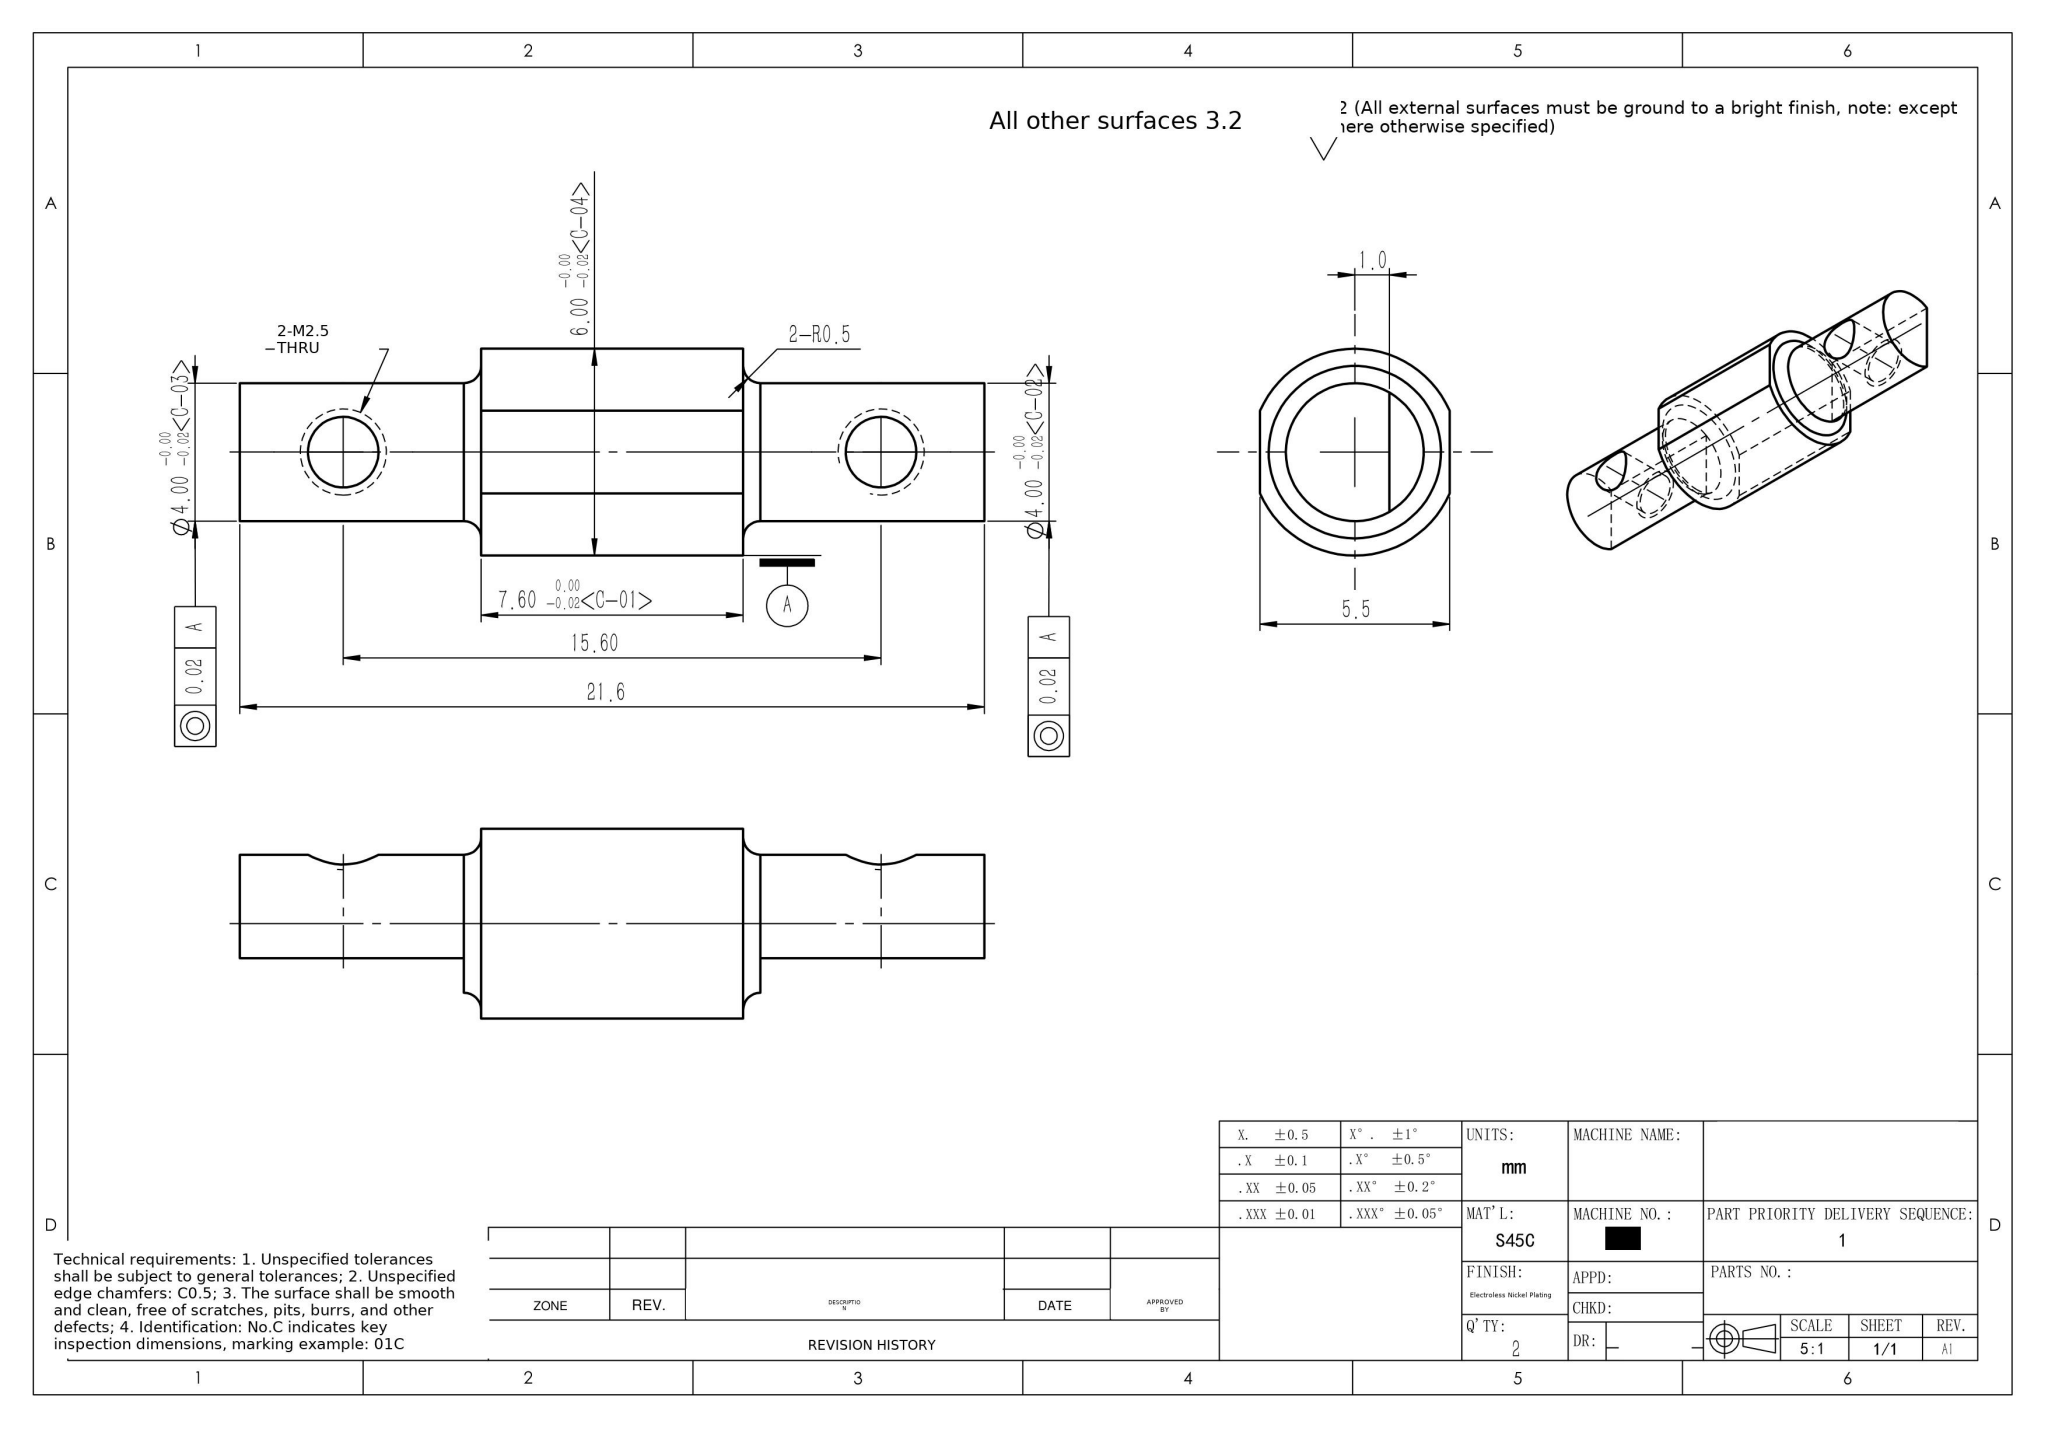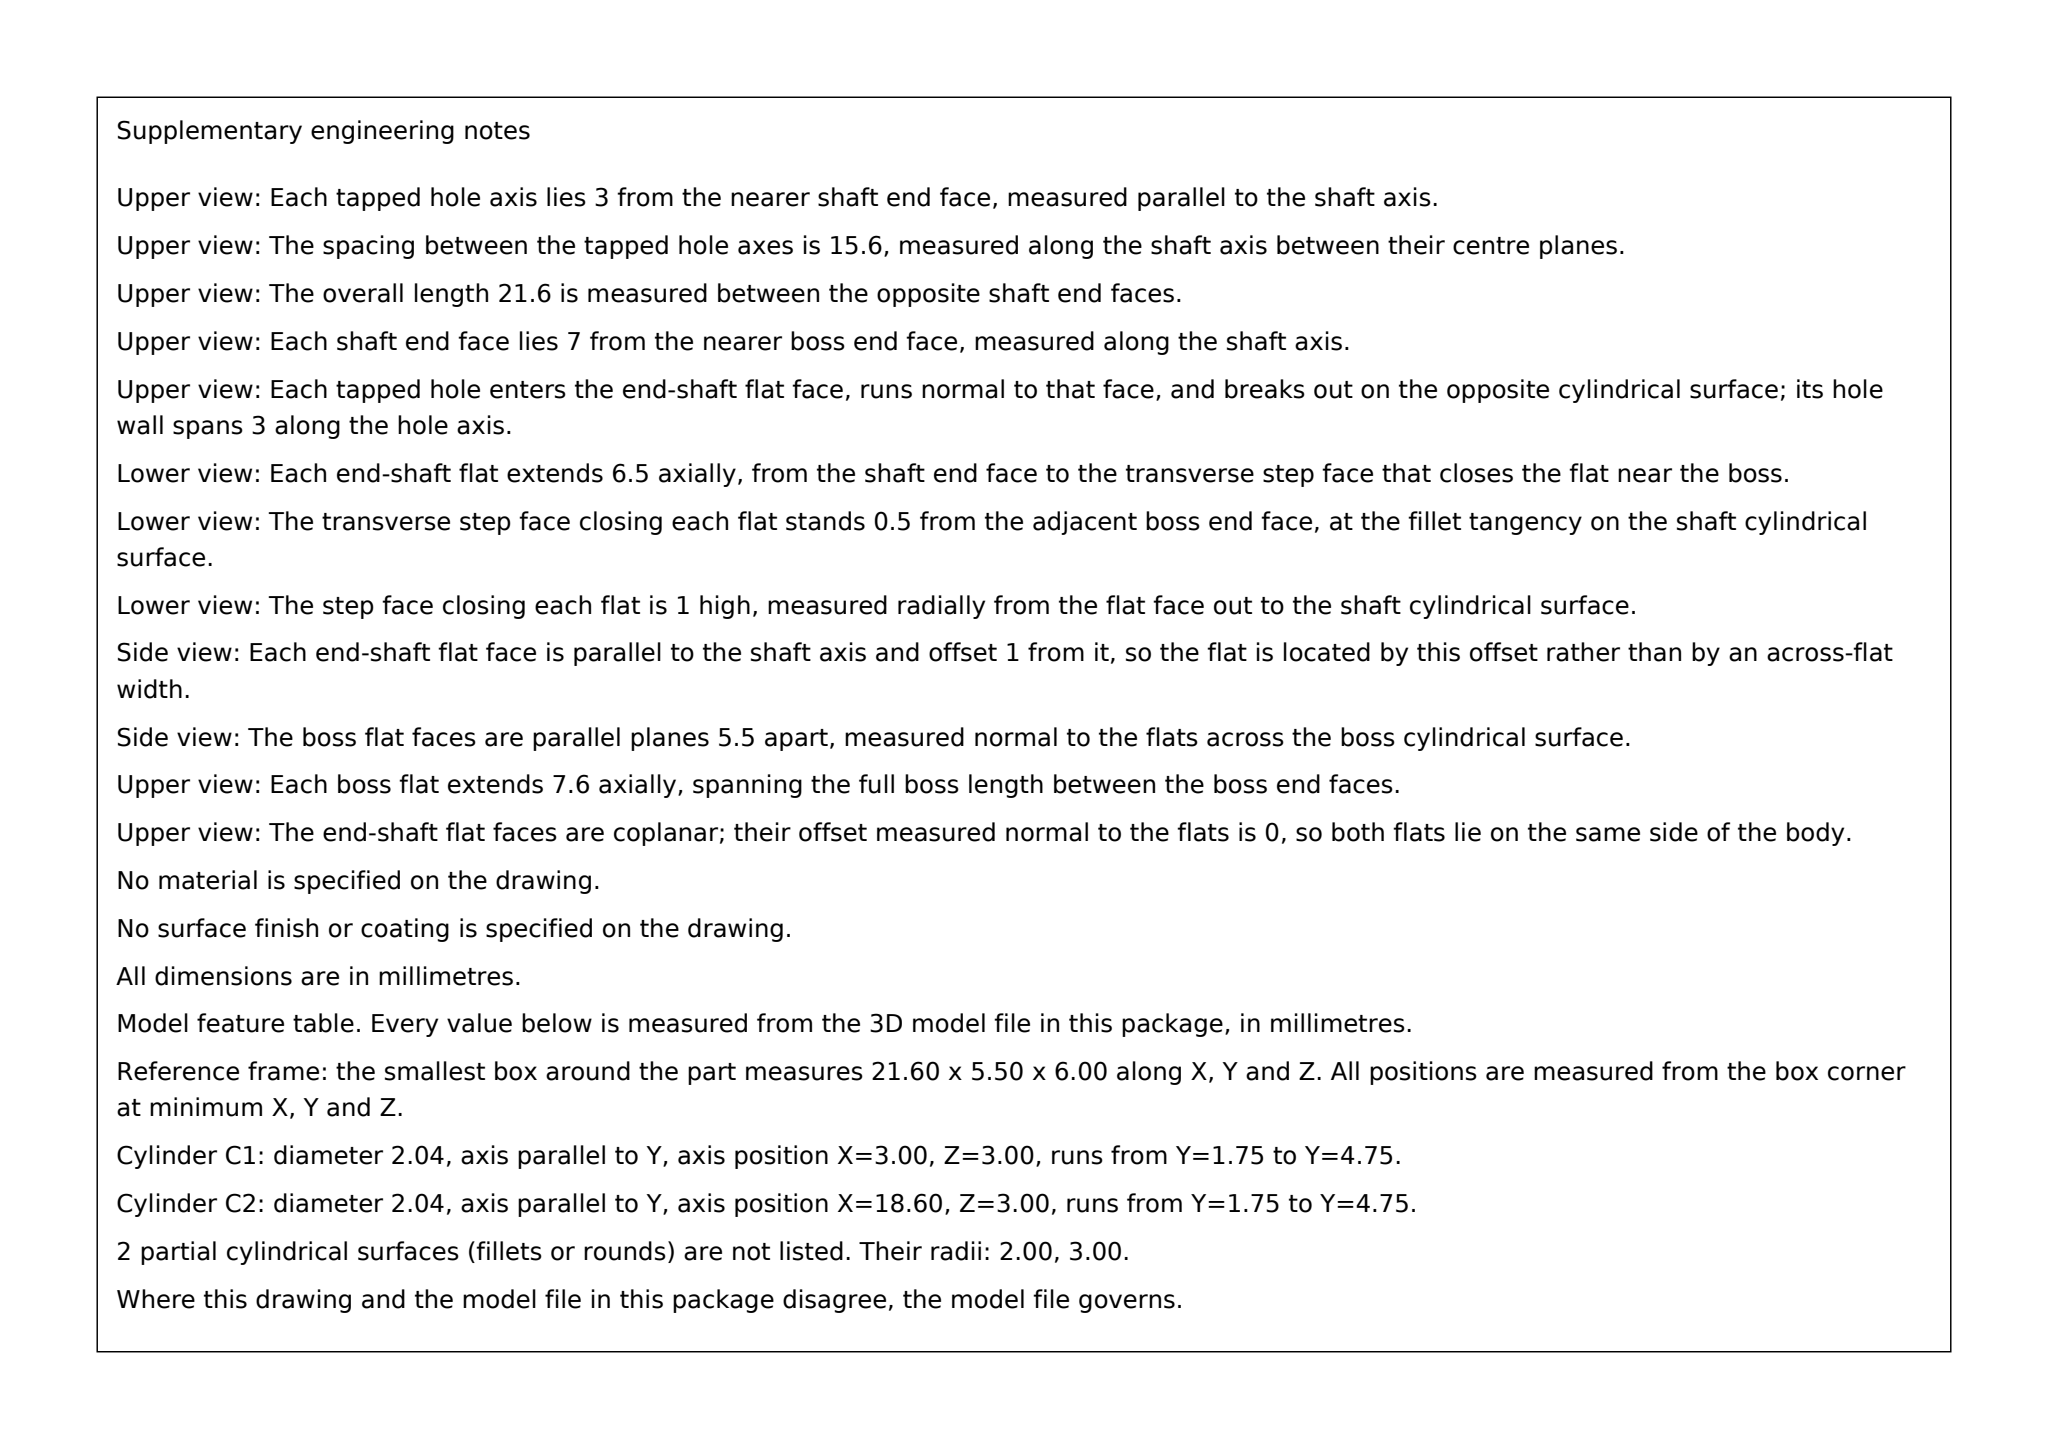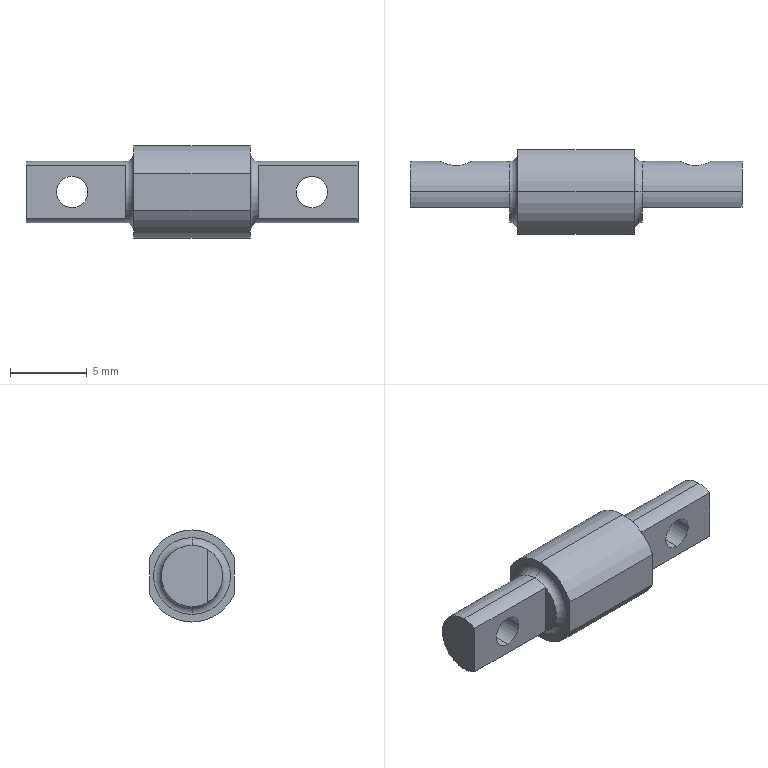Part | SolidWorks | mm | material S45C | 1 solid | 27 faces | box 21.6 x 5.5 x 6 mm | volume 335 mm3 | cylinder 13 | plane 10 | torus 4 | commonest cylinder face diameters 4 x6 2.05 x4 6 x3
Drawing notes:
Ø6.00 CENTRAL BOSS 7.60 LONG, LOCATED 7.00 FROM LEFT END FACE (DATUM X=0) TO NEAR BOSS FACE; FAR FACE AT 14.60. | from the solid: cylinders dia 6.0 axis x length 7.6; axis_planes x=7.0 and x=14.6 (bbox x=0 left end face)
5.5 ACROSS-FLATS ON Ø6.00 BOSS: 2X FLATS EACH 2.75 FROM AXIS, RUNNING FULL BOSS LENGTH 7.60, FROM X=7.00 TO X=14.60. | from the solid: axis_planes y=0.34 and y=5.84 (axis at y=3.09, i.e. ±2.75); boss faces at x=7.0 and 14.6
2X FLAT 1.00 FROM SHAFT AXIS ON THE Ø4.00 END JOURNALS; JOURNALS RUN X=0 TO 6.50 AND X=15.10 TO 21.60 FROM LEFT END FACE. | from the solid: axis_planes y=2.09 count 2 (axis y=3.09, offset 1.00); cylinders dia 4.0 axis x length 6.5; axis_planes x=0, 6.5, 15.1, 21.6
2X M2.5 THRU HOLE AXES LOCATED 3.00 AND 18.60 FROM LEFT END FACE (X=0), PERPENDICULAR TO AND THROUGH SHAFT AXIS. | from the solid: cylinders dia 2.05 axis y at x=3.0 and x=18.6, length 3.0
2X FLAT ON Ø6.00 BOSS, 5.50 ACROSS FLATS, SYMMETRIC ABOUT AXIS; FLATS RUN FULL 7.60 BOSS LENGTH, FROM X=7.00 TO X=14.60 FROM LEFT END FACE | from the solid: axis_planes y=0.34 and y=5.84 (5.50 apart, axis at y=3.09); x planes 7.0 and 14.6; cylinder dia 6.0 axis x length 7.6
2X FLAT ON Ø4.00 SHAFTS, 1.00 FROM AXIS; EACH FLAT RUNS FULL 6.50 SHAFT LENGTH: X=0 TO 6.50 AND X=15.10 TO 21.60 FROM LEFT END FACE | from the solid: axis_planes y=2.09 count 2 (axis y=3.09 → 1.00 offset); cylinders dia 4.0 axis x length 6.5; x planes 0.0, 6.5, 15.1, 21.6
Ø6.00 BOSS AXIAL LOCATION: NEAR FACE 7.00 FROM LEFT END FACE (DATUM A), FAR FACE 14.60; BOSS LENGTH 7.60 | from the solid: x planes at 0.0, 7.0, 14.6; cylinder dia 6.0 axis x length 7.6
4X R0.50 FILLET AT Ø4.00/Ø6.00 SHOULDERS (X=7.00 AND X=14.60) | from the solid: fillet_radii [0.5, 4]; x planes 7.0 and 14.6
2X M2.5 THRU ON SHAFT CENTERLINE, LOCATED 3.00 AND 18.60 FROM LEFT END FACE (DATUM A) | from the solid: cylinders dia 2.05 axis y at x=3.0 and x=18.6, pos z=3.09, length 3.0
4X R0.50 FILLET AT Ø4.00/Ø6.00 SHOULDERS, X=7.00 AND X=14.60 FROM LEFT END FACE (DATUM A) | from the solid: fillet_radii [[0.5, 4]] with axis_planes x=7.0 and x=14.6 at Ø4.00/Ø6.00 cylinder transitions
ALL OTHER SURFACES 3.2 EXCEPT WHERE NOTED | from the solid: no STEP dimension involved; restores text lost by removing garbled surface-finish fragments
build123d program:
from build123d import *

# Parameters (mm, degrees)
SKETCH2_W           = 2.398
SKETCH2_H           = 0.5
CUT_EXTRUDE1_DEPTH  = 7.6
SKETCH5_W           = 8
SKETCH5_H           = 2
CUT_EXTRUDE3_DEPTH  = 6.5
M2_5_TAPPED_HOLE1_D = 2.05


with BuildPart() as part:
    # Sketch1 → Revolve1 (revolve)
    with BuildSketch(Plane.XY, mode=Mode.PRIVATE) as revolve1_sk:
        with BuildLine():
            Line((-10.8, -2), (-4.3, -2))
            ThreePointArc((-4.3, -2), (-3.946, -2.146), (-3.8, -2.5))
            Line((-3.8, -2.5), (-3.8, -3))
            Line((-3.8, -3), (3.8, -3))
            Line((3.8, -3), (3.8, -2.5))
            ThreePointArc((3.8, -2.5), (3.946, -2.146), (4.3, -2))
            Line((4.3, -2), (10.8, -2))
            Line((10.8, -2), (10.8, 0))
            Line((10.8, 0), (-10.8, 0))
            Line((-10.8, 0), (-10.8, -2))
        make_face()
    revolve(revolve1_sk.sketch.rotate(Axis((-6.107, 0, 0), (1, 0, 0)), 270), axis=Axis((-6.107, 0, 0), (1, 0, 0)))

    # Sketch2 → Cut-Extrude1 (cut)
    with BuildSketch(Plane(origin=(3.8, 0, 0), x_dir=(0, 0, -1), z_dir=(1, 0, 0))):
        with Locations((0, 3)):
            Rectangle(SKETCH2_W, SKETCH2_H)
        with Locations((0, -3)):
            Rectangle(SKETCH2_W, SKETCH2_H)
    extrude(amount=-CUT_EXTRUDE1_DEPTH, mode=Mode.SUBTRACT)

    # Sketch5 → Cut-Extrude3 (cut)
    with BuildSketch(Plane(origin=(10.8, 0, 0), x_dir=(0, 0, -1), z_dir=(1, 0, 0))):
        with Locations((0, -2)):
            Rectangle(SKETCH5_W, SKETCH5_H)
    cut_extrude3 = extrude(amount=-CUT_EXTRUDE3_DEPTH, mode=Mode.SUBTRACT)

    # Mirror1: Cut-Extrude3 across plane
    add(cut_extrude3.mirror(Plane(origin=(0, 0, 0), x_dir=(0, 0, 1), z_dir=(1, 0, 0))), mode=Mode.SUBTRACT)

    # M2.5 Tapped Hole1 (through all)
    with Locations(Plane.XZ.offset(1)):
        with Locations((7.8, 0)):
            m2_5_tapped_hole1 = Hole(M2_5_TAPPED_HOLE1_D / 2)

    # Mirror2: M2.5 Tapped Hole1 across plane
    add(m2_5_tapped_hole1.mirror(Plane(origin=(0, 0, 0), x_dir=(0, 0, 1), z_dir=(1, 0, 0))), mode=Mode.SUBTRACT)


solid = part.part